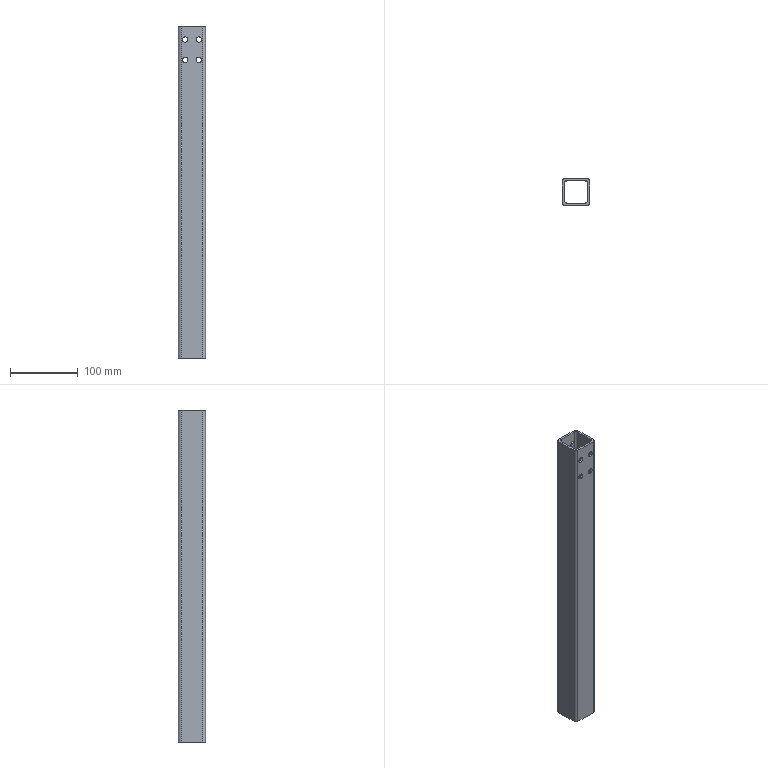Component | NX | VERT_ROD | 1 solid | 26 faces | volume 216353 mm3 | cylinder 16 | plane 10 | commonest cylinder face diameters 8 x16